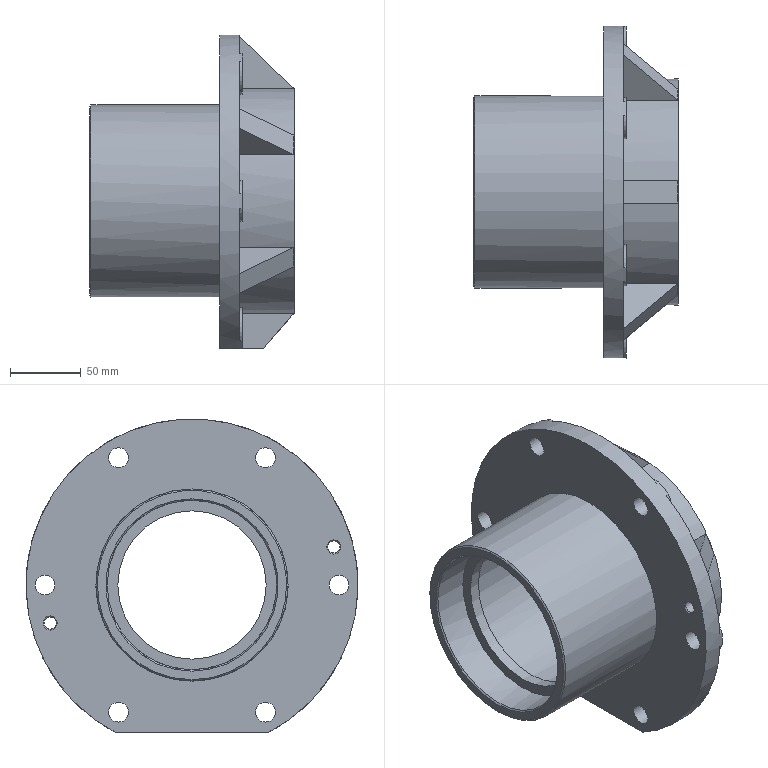Component | NX | FRONT_BEARING_SLEEVE | 1 solid | 84 faces | volume 1225975 mm3 | plane 35 | cylinder 30 | cone 19 | commonest cylinder face diameters 29 x8 8.5 x8 14 x6 120 x2 105 x2 160 x1 136 x1 235 x1